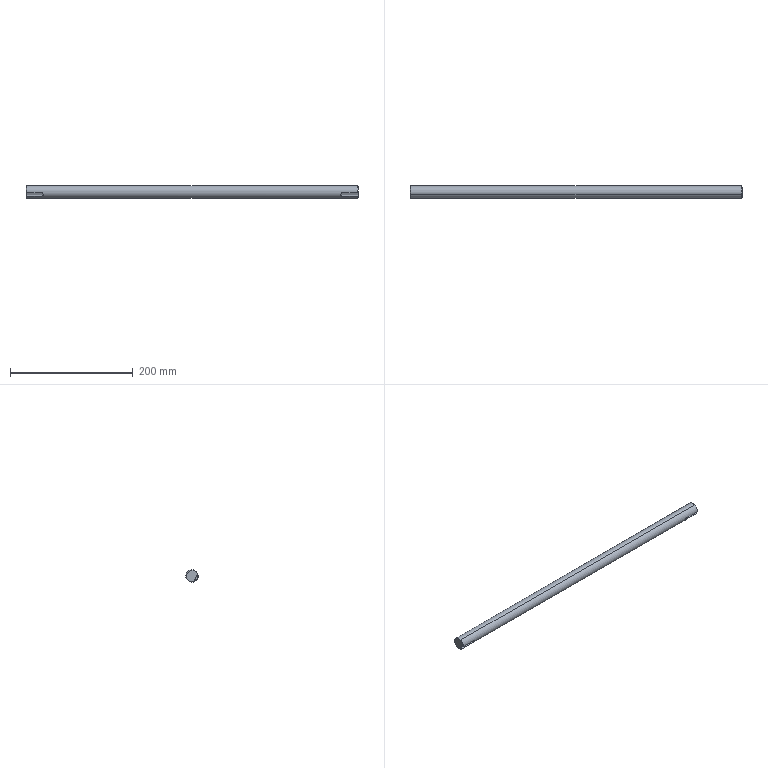Component | SolidWorks | SynchronousAxis-1 | 1 solid | 19 faces | box 540 x 20 x 20 mm | volume 168491 mm3 | plane 8 | cone 6 | cylinder 5 | commonest cylinder face diameters 6 x3 20 x2
build123d program:
from build123d import *

# Parameters (mm, degrees)
SKETCH1_R           = 10
BOSS_EXTRUDE1_DEPTH = 540
CHAMFER1_SIZE       = 1
CUT_EXTRUDE1_DEPTH  = 3.5


with BuildPart() as part:
    # Sketch1 → Boss-Extrude1 (new body)
    with BuildSketch(Plane.XY):
        Circle(SKETCH1_R)
    extrude(amount=BOSS_EXTRUDE1_DEPTH)

    # Chamfer1
    chamfer1_edges = [part.edges().sort_by_distance(p)[0] for p in [
        (-10, 0, 0),
        (-10, 0, 540),
    ]]
    chamfer(chamfer1_edges, length=CHAMFER1_SIZE)

    # Sketch2 → Cut-Extrude1 (cut)
    with BuildSketch(Plane(origin=(0, -10, 0), x_dir=(-1, 0, 0), z_dir=(0, -1, 0))):
        with BuildLine():
            Line((3, 25), (3, -25))
            ThreePointArc((3, -25), (0, -28), (-3, -25))
            Line((-3, -25), (-3, 25))
            ThreePointArc((-3, 25), (0, 28), (3, 25))
        make_face()
    cut_extrude1 = extrude(amount=-CUT_EXTRUDE1_DEPTH, mode=Mode.SUBTRACT)

    # Mirror1: Cut-Extrude1 across plane
    add(cut_extrude1.mirror(Plane.XY.offset(270)), mode=Mode.SUBTRACT)


solid = part.part

# Placed as in the assembly
solid = solid.moved(Location((-244.371, 34.1, 498.836), (24.724, 90, 0)))
STEP:
#1=COLOUR_RGB('',0.7922,0.8196,0.9333);
#2=FILL_AREA_STYLE_COLOUR('',#1);
#3=FILL_AREA_STYLE('',(#2));
#4=SURFACE_STYLE_FILL_AREA(#3);
#5=SURFACE_SIDE_STYLE('',(#4));
#6=SURFACE_STYLE_USAGE(.BOTH.,#5);
#7=PRESENTATION_STYLE_ASSIGNMENT((#6));
#8=CARTESIAN_POINT('',(10.655,1.159,19.425));
#9=VERTEX_POINT('',#8);
#10=CARTESIAN_POINT('',(10.537,1.11,19.532));
#11=VERTEX_POINT('',#10);
#12=CARTESIAN_POINT('',(10.655,1.11,19.532));
#13=DIRECTION('',(-0.,0.9083,0.4182));
#14=DIRECTION('',(1.,0.,0.));
#15=AXIS2_PLACEMENT_3D('',#12,#13,#14);
#16=CIRCLE('',#15,0.1181);
#17=EDGE_CURVE('',#9,#11,#16,.T.);
#18=ORIENTED_EDGE('',*,*,#17,.T.);
#19=CARTESIAN_POINT('',(10.537,0.9849,19.475));
#20=VERTEX_POINT('',#19);
#21=CARTESIAN_POINT('',(10.537,1.11,19.532));
#22=DIRECTION('',(0.,-0.9083,-0.4182));
#23=VECTOR('',#22,39.37);
#24=LINE('',#21,#23);
#25=EDGE_CURVE('',#11,#20,#24,.T.);
#26=ORIENTED_EDGE('',*,*,#25,.T.);
#27=CARTESIAN_POINT('',(10.655,1.051,19.375));
#28=VERTEX_POINT('',#27);
#29=CARTESIAN_POINT('',(10.537,0.9849,19.475));
#30=CARTESIAN_POINT('',(10.537,0.9881,19.467));
#31=CARTESIAN_POINT('',(10.537,0.9917,19.46));
#32=CARTESIAN_POINT('',(10.54,0.9988,19.447));
#33=CARTESIAN_POINT('',(10.543,1.002,19.441));
#34=CARTESIAN_POINT('',(10.549,1.01,19.428));
#35=CARTESIAN_POINT('',(10.552,1.014,19.422));
#36=CARTESIAN_POINT('',(10.561,1.021,19.412));
#37=CARTESIAN_POINT('',(10.566,1.025,19.407));
#38=CARTESIAN_POINT('',(10.577,1.031,19.398));
#39=CARTESIAN_POINT('',(10.583,1.034,19.394));
#40=CARTESIAN_POINT('',(10.595,1.04,19.387));
#41=CARTESIAN_POINT('',(10.602,1.042,19.384));
#42=CARTESIAN_POINT('',(10.616,1.047,19.38));
#43=CARTESIAN_POINT('',(10.624,1.048,19.378));
#44=CARTESIAN_POINT('',(10.639,1.05,19.375));
#45=CARTESIAN_POINT('',(10.647,1.051,19.375));
#46=CARTESIAN_POINT('',(10.655,1.051,19.375));
#47=B_SPLINE_CURVE_WITH_KNOTS('',3,(#29,#30,#31,#32,#33,#34,#35,#36,#37,#38,#39,#40,#41,#42,#43,#44,#45,#46),.UNSPECIFIED.,.F.,.F.,(4,2,2,2,2,2,2,2,4),(0.004718,0.005307,0.005896,0.006485,0.007074,0.007663,0.008252,0.008842,0.009431),.UNSPECIFIED.);
#48=EDGE_CURVE('',#20,#28,#47,.T.);
#49=ORIENTED_EDGE('',*,*,#48,.T.);
#50=CARTESIAN_POINT('',(10.655,1.159,19.425));
#51=DIRECTION('',(0.,-0.9083,-0.4182));
#52=VECTOR('',#51,39.37);
#53=LINE('',#50,#52);
#54=EDGE_CURVE('',#9,#28,#53,.T.);
#55=ORIENTED_EDGE('',*,*,#54,.F.);
#56=EDGE_LOOP('',(#18,#26,#49,#55));
#57=FACE_OUTER_BOUND('',#56,.T.);
#58=CARTESIAN_POINT('',(10.655,1.11,19.532));
#59=DIRECTION('',(0.,-0.9083,-0.4182));
#60=DIRECTION('',(-1.,-0.,0.));
#61=AXIS2_PLACEMENT_3D('',#58,#59,#60);
#62=CYLINDRICAL_SURFACE('',#61,0.1181);
#63=ADVANCED_FACE('',(#57),#62,.F.);
#64=CARTESIAN_POINT('',(-9.621,1.194,19.961));
#65=VERTEX_POINT('',#64);
#66=CARTESIAN_POINT('',(-9.621,1.491,19.317));
#67=VERTEX_POINT('',#66);
#68=CARTESIAN_POINT('',(-9.621,1.343,19.639));
#69=DIRECTION('',(-1.,-0.,0.));
#70=DIRECTION('',(-0.,0.4182,-0.9083));
#71=AXIS2_PLACEMENT_3D('',#68,#69,#70);
#72=CIRCLE('',#71,0.3543);
#73=EDGE_CURVE('',#65,#67,#72,.T.);
#74=ORIENTED_EDGE('',*,*,#73,.F.);
#75=CARTESIAN_POINT('',(-9.582,1.178,19.997));
#76=VERTEX_POINT('',#75);
#77=CARTESIAN_POINT('',(-9.582,1.178,19.997));
#78=DIRECTION('',(0.7071,-0.2957,0.6423));
#79=VECTOR('',#78,39.37);
#80=LINE('',#77,#79);
#81=EDGE_CURVE('',#65,#76,#80,.T.);
#82=ORIENTED_EDGE('',*,*,#81,.T.);
#83=CARTESIAN_POINT('',(-9.582,1.507,19.282));
#84=VERTEX_POINT('',#83);
#85=CARTESIAN_POINT('',(-9.582,1.343,19.639));
#86=DIRECTION('',(1.,0.,-0.));
#87=DIRECTION('',(-0.,0.4182,-0.9083));
#88=AXIS2_PLACEMENT_3D('',#85,#86,#87);
#89=CIRCLE('',#88,0.3937);
#90=EDGE_CURVE('',#84,#76,#89,.T.);
#91=ORIENTED_EDGE('',*,*,#90,.F.);
#92=CARTESIAN_POINT('',(-9.582,1.507,19.282));
#93=DIRECTION('',(0.7071,0.2957,-0.6423));
#94=VECTOR('',#93,39.37);
#95=LINE('',#92,#94);
#96=EDGE_CURVE('',#67,#84,#95,.T.);
#97=ORIENTED_EDGE('',*,*,#96,.F.);
#98=EDGE_LOOP('',(#74,#82,#91,#97));
#99=FACE_OUTER_BOUND('',#98,.T.);
#100=CARTESIAN_POINT('',(-9.582,1.343,19.639));
#101=DIRECTION('',(1.,0.,-0.));
#102=DIRECTION('',(-0.,0.4182,-0.9083));
#103=AXIS2_PLACEMENT_3D('',#100,#101,#102);
#104=CONICAL_SURFACE('',#103,0.3937,0.7854);
#105=ADVANCED_FACE('',(#99),#104,.T.);
#106=CARTESIAN_POINT('',(-9.621,1.088,19.392));
#107=VERTEX_POINT('',#106);
#108=CARTESIAN_POINT('',(-9.621,1.343,19.639));
#109=DIRECTION('',(-1.,-0.,0.));
#110=DIRECTION('',(-0.,0.4182,-0.9083));
#111=AXIS2_PLACEMENT_3D('',#108,#109,#110);
#112=CIRCLE('',#111,0.3543);
#113=EDGE_CURVE('',#67,#107,#112,.T.);
#114=ORIENTED_EDGE('',*,*,#113,.F.);
#115=ORIENTED_EDGE('',*,*,#96,.T.);
#116=CARTESIAN_POINT('',(-9.582,1.051,19.375));
#117=VERTEX_POINT('',#116);
#118=CARTESIAN_POINT('',(-9.582,1.343,19.639));
#119=DIRECTION('',(1.,0.,-0.));
#120=DIRECTION('',(-0.,0.4182,-0.9083));
#121=AXIS2_PLACEMENT_3D('',#118,#119,#120);
#122=CIRCLE('',#121,0.3937);
#123=EDGE_CURVE('',#117,#84,#122,.T.);
#124=ORIENTED_EDGE('',*,*,#123,.F.);
#125=CARTESIAN_POINT('',(-9.621,1.088,19.392));
#126=CARTESIAN_POINT('',(-9.608,1.076,19.386));
#127=CARTESIAN_POINT('',(-9.595,1.063,19.381));
#128=CARTESIAN_POINT('',(-9.582,1.051,19.375));
#129=B_SPLINE_CURVE_WITH_KNOTS('',3,(#125,#126,#127,#128),.UNSPECIFIED.,.F.,.F.,(4,4),(0.005441,0.006894),.UNSPECIFIED.);
#130=EDGE_CURVE('',#107,#117,#129,.T.);
#131=ORIENTED_EDGE('',*,*,#130,.F.);
#132=EDGE_LOOP('',(#114,#115,#124,#131));
#133=FACE_OUTER_BOUND('',#132,.T.);
#134=CARTESIAN_POINT('',(-9.582,1.343,19.639));
#135=DIRECTION('',(1.,0.,-0.));
#136=DIRECTION('',(-0.,0.4182,-0.9083));
#137=AXIS2_PLACEMENT_3D('',#134,#135,#136);
#138=CONICAL_SURFACE('',#137,0.3937,0.7854);
#139=ADVANCED_FACE('',(#133),#138,.T.);
#140=CARTESIAN_POINT('',(11.639,1.491,19.317));
#141=VERTEX_POINT('',#140);
#142=CARTESIAN_POINT('',(11.639,1.194,19.961));
#143=VERTEX_POINT('',#142);
#144=CARTESIAN_POINT('',(11.639,1.343,19.639));
#145=DIRECTION('',(1.,0.,-0.));
#146=DIRECTION('',(0.,0.4182,-0.9083));
#147=AXIS2_PLACEMENT_3D('',#144,#145,#146);
#148=CIRCLE('',#147,0.3543);
#149=EDGE_CURVE('',#141,#143,#148,.T.);
#150=ORIENTED_EDGE('',*,*,#149,.F.);
#151=CARTESIAN_POINT('',(11.6,1.507,19.282));
#152=VERTEX_POINT('',#151);
#153=CARTESIAN_POINT('',(11.639,1.491,19.317));
#154=DIRECTION('',(-0.7071,0.2957,-0.6423));
#155=VECTOR('',#154,39.37);
#156=LINE('',#153,#155);
#157=EDGE_CURVE('',#141,#152,#156,.T.);
#158=ORIENTED_EDGE('',*,*,#157,.T.);
#159=CARTESIAN_POINT('',(11.6,1.178,19.997));
#160=VERTEX_POINT('',#159);
#161=CARTESIAN_POINT('',(11.6,1.343,19.639));
#162=DIRECTION('',(-1.,-0.,0.));
#163=DIRECTION('',(0.,0.4182,-0.9083));
#164=AXIS2_PLACEMENT_3D('',#161,#162,#163);
#165=CIRCLE('',#164,0.3937);
#166=EDGE_CURVE('',#160,#152,#165,.T.);
#167=ORIENTED_EDGE('',*,*,#166,.F.);
#168=CARTESIAN_POINT('',(11.639,1.194,19.961));
#169=DIRECTION('',(-0.7071,-0.2957,0.6423));
#170=VECTOR('',#169,39.37);
#171=LINE('',#168,#170);
#172=EDGE_CURVE('',#143,#160,#171,.T.);
#173=ORIENTED_EDGE('',*,*,#172,.F.);
#174=EDGE_LOOP('',(#150,#158,#167,#173));
#175=FACE_OUTER_BOUND('',#174,.T.);
#176=CARTESIAN_POINT('',(11.639,1.343,19.639));
#177=DIRECTION('',(-1.,-0.,0.));
#178=DIRECTION('',(0.,-0.4182,0.9083));
#179=AXIS2_PLACEMENT_3D('',#176,#177,#178);
#180=CONICAL_SURFACE('',#179,0.3543,0.7854);
#181=ADVANCED_FACE('',(#175),#180,.T.);
#182=CARTESIAN_POINT('',(11.639,0.9897,19.607));
#183=VERTEX_POINT('',#182);
#184=CARTESIAN_POINT('',(11.639,1.343,19.639));
#185=DIRECTION('',(1.,0.,-0.));
#186=DIRECTION('',(0.,0.4182,-0.9083));
#187=AXIS2_PLACEMENT_3D('',#184,#185,#186);
#188=CIRCLE('',#187,0.3543);
#189=EDGE_CURVE('',#143,#183,#188,.T.);
#190=ORIENTED_EDGE('',*,*,#189,.F.);
#191=ORIENTED_EDGE('',*,*,#172,.T.);
#192=CARTESIAN_POINT('',(11.6,0.952,19.589));
#193=VERTEX_POINT('',#192);
#194=CARTESIAN_POINT('',(11.6,1.343,19.639));
#195=DIRECTION('',(-1.,-0.,0.));
#196=DIRECTION('',(0.,0.4182,-0.9083));
#197=AXIS2_PLACEMENT_3D('',#194,#195,#196);
#198=CIRCLE('',#197,0.3937);
#199=EDGE_CURVE('',#193,#160,#198,.T.);
#200=ORIENTED_EDGE('',*,*,#199,.F.);
#201=CARTESIAN_POINT('',(11.6,0.952,19.589));
#202=CARTESIAN_POINT('',(11.613,0.9645,19.595));
#203=CARTESIAN_POINT('',(11.626,0.9771,19.601));
#204=CARTESIAN_POINT('',(11.639,0.9897,19.607));
#205=B_SPLINE_CURVE_WITH_KNOTS('',3,(#201,#202,#203,#204),.UNSPECIFIED.,.F.,.F.,(4,4),(0.005238,0.006691),.UNSPECIFIED.);
#206=EDGE_CURVE('',#193,#183,#205,.T.);
#207=ORIENTED_EDGE('',*,*,#206,.T.);
#208=EDGE_LOOP('',(#190,#191,#200,#207));
#209=FACE_OUTER_BOUND('',#208,.T.);
#210=CARTESIAN_POINT('',(11.639,1.343,19.639));
#211=DIRECTION('',(-1.,-0.,0.));
#212=DIRECTION('',(0.,-0.4182,0.9083));
#213=AXIS2_PLACEMENT_3D('',#210,#211,#212);
#214=CONICAL_SURFACE('',#213,0.3543,0.7854);
#215=ADVANCED_FACE('',(#209),#214,.T.);
#216=ORIENTED_EDGE('',*,*,#166,.T.);
#217=CARTESIAN_POINT('',(11.639,1.507,19.282));
#218=DIRECTION('',(-1.,-0.,0.));
#219=VECTOR('',#218,39.37);
#220=LINE('',#217,#219);
#221=EDGE_CURVE('',#152,#84,#220,.T.);
#222=ORIENTED_EDGE('',*,*,#221,.T.);
#223=ORIENTED_EDGE('',*,*,#90,.T.);
#224=CARTESIAN_POINT('',(11.639,1.178,19.997));
#225=DIRECTION('',(-1.,-0.,0.));
#226=VECTOR('',#225,39.37);
#227=LINE('',#224,#226);
#228=EDGE_CURVE('',#160,#76,#227,.T.);
#229=ORIENTED_EDGE('',*,*,#228,.F.);
#230=EDGE_LOOP('',(#216,#222,#223,#229));
#231=FACE_OUTER_BOUND('',#230,.T.);
#232=CARTESIAN_POINT('',(11.639,1.343,19.639));
#233=DIRECTION('',(-1.,-0.,0.));
#234=DIRECTION('',(0.,-0.4182,0.9083));
#235=AXIS2_PLACEMENT_3D('',#232,#233,#234);
#236=CYLINDRICAL_SURFACE('',#235,0.3937);
#237=ADVANCED_FACE('',(#231),#236,.T.);
#238=ORIENTED_EDGE('',*,*,#221,.F.);
#239=CARTESIAN_POINT('',(11.6,1.051,19.375));
#240=VERTEX_POINT('',#239);
#241=CARTESIAN_POINT('',(11.6,1.343,19.639));
#242=DIRECTION('',(-1.,-0.,0.));
#243=DIRECTION('',(0.,0.4182,-0.9083));
#244=AXIS2_PLACEMENT_3D('',#241,#242,#243);
#245=CIRCLE('',#244,0.3937);
#246=EDGE_CURVE('',#152,#240,#245,.T.);
#247=ORIENTED_EDGE('',*,*,#246,.T.);
#248=CARTESIAN_POINT('',(11.639,1.051,19.375));
#249=DIRECTION('',(1.,0.,-0.));
#250=VECTOR('',#249,39.37);
#251=LINE('',#248,#250);
#252=EDGE_CURVE('',#28,#240,#251,.T.);
#253=ORIENTED_EDGE('',*,*,#252,.F.);
#254=ORIENTED_EDGE('',*,*,#48,.F.);
#255=CARTESIAN_POINT('',(10.655,0.952,19.589));
#256=VERTEX_POINT('',#255);
#257=CARTESIAN_POINT('',(10.655,0.952,19.589));
#258=CARTESIAN_POINT('',(10.647,0.952,19.589));
#259=CARTESIAN_POINT('',(10.639,0.9521,19.589));
#260=CARTESIAN_POINT('',(10.624,0.9525,19.585));
#261=CARTESIAN_POINT('',(10.616,0.9528,19.583));
#262=CARTESIAN_POINT('',(10.602,0.9538,19.577));
#263=CARTESIAN_POINT('',(10.595,0.9544,19.573));
#264=CARTESIAN_POINT('',(10.583,0.9559,19.565));
#265=CARTESIAN_POINT('',(10.577,0.9569,19.56));
#266=CARTESIAN_POINT('',(10.56,0.9605,19.543));
#267=CARTESIAN_POINT('',(10.552,0.9639,19.53));
#268=CARTESIAN_POINT('',(10.543,0.9705,19.51));
#269=CARTESIAN_POINT('',(10.54,0.9731,19.503));
#270=CARTESIAN_POINT('',(10.537,0.9786,19.489));
#271=CARTESIAN_POINT('',(10.537,0.9817,19.482));
#272=CARTESIAN_POINT('',(10.537,0.9849,19.475));
#273=B_SPLINE_CURVE_WITH_KNOTS('',3,(#257,#258,#259,#260,#261,#262,#263,#264,#265,#266,#267,#268,#269,#270,#271,#272),.UNSPECIFIED.,.F.,.F.,(4,2,2,2,2,2,2,4),(0.,0.0005898,0.00118,0.001769,0.002359,0.003539,0.004128,0.004718),.UNSPECIFIED.);
#274=EDGE_CURVE('',#256,#20,#273,.T.);
#275=ORIENTED_EDGE('',*,*,#274,.F.);
#276=CARTESIAN_POINT('',(11.639,0.952,19.589));
#277=DIRECTION('',(-1.,-0.,0.));
#278=VECTOR('',#277,39.37);
#279=LINE('',#276,#278);
#280=EDGE_CURVE('',#193,#256,#279,.T.);
#281=ORIENTED_EDGE('',*,*,#280,.F.);
#282=ORIENTED_EDGE('',*,*,#199,.T.);
#283=ORIENTED_EDGE('',*,*,#228,.T.);
#284=CARTESIAN_POINT('',(-9.582,0.952,19.589));
#285=VERTEX_POINT('',#284);
#286=CARTESIAN_POINT('',(-9.582,1.343,19.639));
#287=DIRECTION('',(1.,0.,-0.));
#288=DIRECTION('',(-0.,0.4182,-0.9083));
#289=AXIS2_PLACEMENT_3D('',#286,#287,#288);
#290=CIRCLE('',#289,0.3937);
#291=EDGE_CURVE('',#76,#285,#290,.T.);
#292=ORIENTED_EDGE('',*,*,#291,.T.);
#293=CARTESIAN_POINT('',(-8.637,0.952,19.589));
#294=VERTEX_POINT('',#293);
#295=CARTESIAN_POINT('',(11.639,0.952,19.589));
#296=DIRECTION('',(1.,0.,-0.));
#297=VECTOR('',#296,39.37);
#298=LINE('',#295,#297);
#299=EDGE_CURVE('',#285,#294,#298,.T.);
#300=ORIENTED_EDGE('',*,*,#299,.T.);
#301=CARTESIAN_POINT('',(-8.637,1.051,19.375));
#302=VERTEX_POINT('',#301);
#303=CARTESIAN_POINT('',(-8.637,0.952,19.589));
#304=CARTESIAN_POINT('',(-8.629,0.952,19.589));
#305=CARTESIAN_POINT('',(-8.621,0.9521,19.589));
#306=CARTESIAN_POINT('',(-8.606,0.9525,19.585));
#307=CARTESIAN_POINT('',(-8.598,0.9528,19.583));
#308=CARTESIAN_POINT('',(-8.584,0.9538,19.577));
#309=CARTESIAN_POINT('',(-8.577,0.9544,19.573));
#310=CARTESIAN_POINT('',(-8.565,0.9559,19.565));
#311=CARTESIAN_POINT('',(-8.559,0.9569,19.56));
#312=CARTESIAN_POINT('',(-8.542,0.9605,19.543));
#313=CARTESIAN_POINT('',(-8.534,0.9639,19.53));
#314=CARTESIAN_POINT('',(-8.525,0.9705,19.51));
#315=CARTESIAN_POINT('',(-8.522,0.973,19.503));
#316=CARTESIAN_POINT('',(-8.519,0.9786,19.489));
#317=CARTESIAN_POINT('',(-8.519,0.9816,19.482));
#318=CARTESIAN_POINT('',(-8.519,0.9881,19.468));
#319=CARTESIAN_POINT('',(-8.519,0.9916,19.461));
#320=CARTESIAN_POINT('',(-8.522,0.9988,19.447));
#321=CARTESIAN_POINT('',(-8.525,1.002,19.441));
#322=CARTESIAN_POINT('',(-8.531,1.01,19.428));
#323=CARTESIAN_POINT('',(-8.534,1.014,19.423));
#324=CARTESIAN_POINT('',(-8.543,1.021,19.412));
#325=CARTESIAN_POINT('',(-8.548,1.025,19.407));
#326=CARTESIAN_POINT('',(-8.559,1.031,19.398));
#327=CARTESIAN_POINT('',(-8.564,1.034,19.394));
#328=CARTESIAN_POINT('',(-8.577,1.04,19.387));
#329=CARTESIAN_POINT('',(-8.584,1.042,19.384));
#330=CARTESIAN_POINT('',(-8.598,1.047,19.38));
#331=CARTESIAN_POINT('',(-8.606,1.048,19.378));
#332=CARTESIAN_POINT('',(-8.621,1.05,19.375));
#333=CARTESIAN_POINT('',(-8.629,1.051,19.375));
#334=CARTESIAN_POINT('',(-8.637,1.051,19.375));
#335=B_SPLINE_CURVE_WITH_KNOTS('',3,(#303,#304,#305,#306,#307,#308,#309,#310,#311,#312,#313,#314,#315,#316,#317,#318,#319,#320,#321,#322,#323,#324,#325,#326,#327,#328,#329,#330,#331,#332,#333,#334),.UNSPECIFIED.,.F.,.F.,(4,2,2,2,2,2,2,2,2,2,2,2,2,2,2,4),(0.,0.0005894,0.001179,0.001768,0.002358,0.003536,0.004126,0.004715,0.005305,0.005894,0.006484,0.007073,0.007662,0.008252,0.008841,0.009431),.UNSPECIFIED.);
#336=EDGE_CURVE('',#294,#302,#335,.T.);
#337=ORIENTED_EDGE('',*,*,#336,.T.);
#338=CARTESIAN_POINT('',(11.639,1.051,19.375));
#339=DIRECTION('',(-1.,-0.,0.));
#340=VECTOR('',#339,39.37);
#341=LINE('',#338,#340);
#342=EDGE_CURVE('',#302,#117,#341,.T.);
#343=ORIENTED_EDGE('',*,*,#342,.T.);
#344=ORIENTED_EDGE('',*,*,#123,.T.);
#345=EDGE_LOOP('',(#238,#247,#253,#254,#275,#281,#282,#283,#292,#300,#337,#343,#344));
#346=FACE_OUTER_BOUND('',#345,.T.);
#347=CARTESIAN_POINT('',(11.639,1.343,19.639));
#348=DIRECTION('',(-1.,-0.,0.));
#349=DIRECTION('',(0.,-0.4182,0.9083));
#350=AXIS2_PLACEMENT_3D('',#347,#348,#349);
#351=CYLINDRICAL_SURFACE('',#350,0.3937);
#352=ADVANCED_FACE('',(#346),#351,.T.);
#353=CARTESIAN_POINT('',(11.639,1.061,19.639));
#354=VERTEX_POINT('',#353);
#355=CARTESIAN_POINT('',(11.639,1.159,19.425));
#356=VERTEX_POINT('',#355);
#357=CARTESIAN_POINT('',(11.639,1.11,19.532));
#358=DIRECTION('',(-0.,0.4182,-0.9083));
#359=VECTOR('',#358,39.37);
#360=LINE('',#357,#359);
#361=EDGE_CURVE('',#354,#356,#360,.T.);
#362=ORIENTED_EDGE('',*,*,#361,.T.);
#363=CARTESIAN_POINT('',(11.639,1.088,19.392));
#364=VERTEX_POINT('',#363);
#365=CARTESIAN_POINT('',(11.639,1.392,19.532));
#366=DIRECTION('',(0.,-0.9083,-0.4182));
#367=VECTOR('',#366,39.37);
#368=LINE('',#365,#367);
#369=EDGE_CURVE('',#356,#364,#368,.T.);
#370=ORIENTED_EDGE('',*,*,#369,.T.);
#371=CARTESIAN_POINT('',(11.639,1.343,19.639));
#372=DIRECTION('',(1.,0.,-0.));
#373=DIRECTION('',(0.,0.4182,-0.9083));
#374=AXIS2_PLACEMENT_3D('',#371,#372,#373);
#375=CIRCLE('',#374,0.3543);
#376=EDGE_CURVE('',#364,#141,#375,.T.);
#377=ORIENTED_EDGE('',*,*,#376,.T.);
#378=ORIENTED_EDGE('',*,*,#149,.T.);
#379=ORIENTED_EDGE('',*,*,#189,.T.);
#380=CARTESIAN_POINT('',(11.639,1.293,19.746));
#381=DIRECTION('',(-0.,0.9083,0.4182));
#382=VECTOR('',#381,39.37);
#383=LINE('',#380,#382);
#384=EDGE_CURVE('',#183,#354,#383,.T.);
#385=ORIENTED_EDGE('',*,*,#384,.T.);
#386=EDGE_LOOP('',(#362,#370,#377,#378,#379,#385));
#387=FACE_OUTER_BOUND('',#386,.T.);
#388=CARTESIAN_POINT('',(11.639,1.343,19.639));
#389=DIRECTION('',(1.,0.,-0.));
#390=DIRECTION('',(-0.,0.4182,-0.9083));
#391=AXIS2_PLACEMENT_3D('',#388,#389,#390);
#392=PLANE('',#391);
#393=ADVANCED_FACE('',(#387),#392,.T.);
#394=ORIENTED_EDGE('',*,*,#157,.F.);
#395=ORIENTED_EDGE('',*,*,#376,.F.);
#396=CARTESIAN_POINT('',(11.639,1.088,19.392));
#397=CARTESIAN_POINT('',(11.626,1.076,19.386));
#398=CARTESIAN_POINT('',(11.613,1.063,19.381));
#399=CARTESIAN_POINT('',(11.6,1.051,19.375));
#400=B_SPLINE_CURVE_WITH_KNOTS('',3,(#396,#397,#398,#399),.UNSPECIFIED.,.F.,.F.,(4,4),(0.005441,0.006894),.UNSPECIFIED.);
#401=EDGE_CURVE('',#364,#240,#400,.T.);
#402=ORIENTED_EDGE('',*,*,#401,.T.);
#403=ORIENTED_EDGE('',*,*,#246,.F.);
#404=EDGE_LOOP('',(#394,#395,#402,#403));
#405=FACE_OUTER_BOUND('',#404,.T.);
#406=CARTESIAN_POINT('',(11.639,1.343,19.639));
#407=DIRECTION('',(-1.,-0.,0.));
#408=DIRECTION('',(0.,-0.4182,0.9083));
#409=AXIS2_PLACEMENT_3D('',#406,#407,#408);
#410=CONICAL_SURFACE('',#409,0.3543,0.7854);
#411=ADVANCED_FACE('',(#405),#410,.T.);
#412=CARTESIAN_POINT('',(-9.621,1.061,19.639));
#413=VERTEX_POINT('',#412);
#414=CARTESIAN_POINT('',(-9.621,1.159,19.425));
#415=VERTEX_POINT('',#414);
#416=CARTESIAN_POINT('',(-9.621,1.11,19.532));
#417=DIRECTION('',(-0.,0.4182,-0.9083));
#418=VECTOR('',#417,39.37);
#419=LINE('',#416,#418);
#420=EDGE_CURVE('',#413,#415,#419,.T.);
#421=ORIENTED_EDGE('',*,*,#420,.F.);
#422=CARTESIAN_POINT('',(-9.621,0.9897,19.607));
#423=VERTEX_POINT('',#422);
#424=CARTESIAN_POINT('',(-9.621,1.293,19.746));
#425=DIRECTION('',(0.,-0.9083,-0.4182));
#426=VECTOR('',#425,39.37);
#427=LINE('',#424,#426);
#428=EDGE_CURVE('',#413,#423,#427,.T.);
#429=ORIENTED_EDGE('',*,*,#428,.T.);
#430=CARTESIAN_POINT('',(-9.621,1.343,19.639));
#431=DIRECTION('',(-1.,-0.,0.));
#432=DIRECTION('',(-0.,0.4182,-0.9083));
#433=AXIS2_PLACEMENT_3D('',#430,#431,#432);
#434=CIRCLE('',#433,0.3543);
#435=EDGE_CURVE('',#423,#65,#434,.T.);
#436=ORIENTED_EDGE('',*,*,#435,.T.);
#437=ORIENTED_EDGE('',*,*,#73,.T.);
#438=ORIENTED_EDGE('',*,*,#113,.T.);
#439=CARTESIAN_POINT('',(-9.621,1.392,19.532));
#440=DIRECTION('',(-0.,0.9083,0.4182));
#441=VECTOR('',#440,39.37);
#442=LINE('',#439,#441);
#443=EDGE_CURVE('',#107,#415,#442,.T.);
#444=ORIENTED_EDGE('',*,*,#443,.T.);
#445=EDGE_LOOP('',(#421,#429,#436,#437,#438,#444));
#446=FACE_OUTER_BOUND('',#445,.T.);
#447=CARTESIAN_POINT('',(-9.621,1.343,19.639));
#448=DIRECTION('',(1.,0.,-0.));
#449=DIRECTION('',(-0.,0.4182,-0.9083));
#450=AXIS2_PLACEMENT_3D('',#447,#448,#449);
#451=PLANE('',#450);
#452=ADVANCED_FACE('',(#446),#451,.F.);
#453=ORIENTED_EDGE('',*,*,#81,.F.);
#454=ORIENTED_EDGE('',*,*,#435,.F.);
#455=CARTESIAN_POINT('',(-9.582,0.952,19.589));
#456=CARTESIAN_POINT('',(-9.595,0.9645,19.595));
#457=CARTESIAN_POINT('',(-9.608,0.9771,19.601));
#458=CARTESIAN_POINT('',(-9.621,0.9897,19.607));
#459=B_SPLINE_CURVE_WITH_KNOTS('',3,(#455,#456,#457,#458),.UNSPECIFIED.,.F.,.F.,(4,4),(0.005238,0.006691),.UNSPECIFIED.);
#460=EDGE_CURVE('',#285,#423,#459,.T.);
#461=ORIENTED_EDGE('',*,*,#460,.F.);
#462=ORIENTED_EDGE('',*,*,#291,.F.);
#463=EDGE_LOOP('',(#453,#454,#461,#462));
#464=FACE_OUTER_BOUND('',#463,.T.);
#465=CARTESIAN_POINT('',(-9.582,1.343,19.639));
#466=DIRECTION('',(1.,0.,-0.));
#467=DIRECTION('',(-0.,0.4182,-0.9083));
#468=AXIS2_PLACEMENT_3D('',#465,#466,#467);
#469=CONICAL_SURFACE('',#468,0.3937,0.7854);
#470=ADVANCED_FACE('',(#464),#469,.T.);
#471=CARTESIAN_POINT('',(-8.637,1.061,19.639));
#472=VERTEX_POINT('',#471);
#473=CARTESIAN_POINT('',(-8.637,1.061,19.639));
#474=DIRECTION('',(0.,-0.9083,-0.4182));
#475=VECTOR('',#474,39.37);
#476=LINE('',#473,#475);
#477=EDGE_CURVE('',#472,#294,#476,.T.);
#478=ORIENTED_EDGE('',*,*,#477,.F.);
#479=CARTESIAN_POINT('',(-8.637,1.159,19.425));
#480=VERTEX_POINT('',#479);
#481=CARTESIAN_POINT('',(-8.637,1.11,19.532));
#482=DIRECTION('',(0.,-0.9083,-0.4182));
#483=DIRECTION('',(-1.,-0.,0.));
#484=AXIS2_PLACEMENT_3D('',#481,#482,#483);
#485=CIRCLE('',#484,0.1181);
#486=EDGE_CURVE('',#480,#472,#485,.T.);
#487=ORIENTED_EDGE('',*,*,#486,.F.);
#488=CARTESIAN_POINT('',(-8.637,1.159,19.425));
#489=DIRECTION('',(0.,-0.9083,-0.4182));
#490=VECTOR('',#489,39.37);
#491=LINE('',#488,#490);
#492=EDGE_CURVE('',#480,#302,#491,.T.);
#493=ORIENTED_EDGE('',*,*,#492,.T.);
#494=ORIENTED_EDGE('',*,*,#336,.F.);
#495=EDGE_LOOP('',(#478,#487,#493,#494));
#496=FACE_OUTER_BOUND('',#495,.T.);
#497=CARTESIAN_POINT('',(-8.637,1.11,19.532));
#498=DIRECTION('',(0.,-0.9083,-0.4182));
#499=DIRECTION('',(-1.,-0.,0.));
#500=AXIS2_PLACEMENT_3D('',#497,#498,#499);
#501=CYLINDRICAL_SURFACE('',#500,0.1181);
#502=ADVANCED_FACE('',(#496),#501,.F.);
#503=ORIENTED_EDGE('',*,*,#420,.T.);
#504=CARTESIAN_POINT('',(-10.605,1.159,19.425));
#505=DIRECTION('',(1.,0.,0.));
#506=VECTOR('',#505,39.37);
#507=LINE('',#504,#506);
#508=EDGE_CURVE('',#415,#480,#507,.T.);
#509=ORIENTED_EDGE('',*,*,#508,.T.);
#510=ORIENTED_EDGE('',*,*,#486,.T.);
#511=CARTESIAN_POINT('',(-10.605,1.061,19.639));
#512=DIRECTION('',(-1.,-0.,-0.));
#513=VECTOR('',#512,39.37);
#514=LINE('',#511,#513);
#515=EDGE_CURVE('',#472,#413,#514,.T.);
#516=ORIENTED_EDGE('',*,*,#515,.T.);
#517=EDGE_LOOP('',(#503,#509,#510,#516));
#518=FACE_OUTER_BOUND('',#517,.T.);
#519=CARTESIAN_POINT('',(-10.605,1.11,19.532));
#520=DIRECTION('',(0.,-0.9083,-0.4182));
#521=DIRECTION('',(-1.,-0.,0.));
#522=AXIS2_PLACEMENT_3D('',#519,#520,#521);
#523=PLANE('',#522);
#524=ADVANCED_FACE('',(#518),#523,.T.);
#525=ORIENTED_EDGE('',*,*,#460,.T.);
#526=ORIENTED_EDGE('',*,*,#428,.F.);
#527=ORIENTED_EDGE('',*,*,#515,.F.);
#528=ORIENTED_EDGE('',*,*,#477,.T.);
#529=ORIENTED_EDGE('',*,*,#299,.F.);
#530=EDGE_LOOP('',(#525,#526,#527,#528,#529));
#531=FACE_OUTER_BOUND('',#530,.T.);
#532=CARTESIAN_POINT('',(-10.605,1.061,19.639));
#533=DIRECTION('',(0.,-0.4182,0.9083));
#534=DIRECTION('',(1.,0.,0.));
#535=AXIS2_PLACEMENT_3D('',#532,#533,#534);
#536=PLANE('',#535);
#537=ADVANCED_FACE('',(#531),#536,.F.);
#538=ORIENTED_EDGE('',*,*,#492,.F.);
#539=ORIENTED_EDGE('',*,*,#508,.F.);
#540=ORIENTED_EDGE('',*,*,#443,.F.);
#541=ORIENTED_EDGE('',*,*,#130,.T.);
#542=ORIENTED_EDGE('',*,*,#342,.F.);
#543=EDGE_LOOP('',(#538,#539,#540,#541,#542));
#544=FACE_OUTER_BOUND('',#543,.T.);
#545=CARTESIAN_POINT('',(-10.605,1.159,19.425));
#546=DIRECTION('',(-0.,0.4182,-0.9083));
#547=DIRECTION('',(-1.,-0.,-0.));
#548=AXIS2_PLACEMENT_3D('',#545,#546,#547);
#549=PLANE('',#548);
#550=ADVANCED_FACE('',(#544),#549,.F.);
#551=ORIENTED_EDGE('',*,*,#25,.F.);
#552=CARTESIAN_POINT('',(10.655,1.061,19.639));
#553=VERTEX_POINT('',#552);
#554=CARTESIAN_POINT('',(10.655,1.11,19.532));
#555=DIRECTION('',(-0.,0.9083,0.4182));
#556=DIRECTION('',(1.,0.,0.));
#557=AXIS2_PLACEMENT_3D('',#554,#555,#556);
#558=CIRCLE('',#557,0.1181);
#559=EDGE_CURVE('',#11,#553,#558,.T.);
#560=ORIENTED_EDGE('',*,*,#559,.T.);
#561=CARTESIAN_POINT('',(10.655,1.061,19.639));
#562=DIRECTION('',(0.,-0.9083,-0.4182));
#563=VECTOR('',#562,39.37);
#564=LINE('',#561,#563);
#565=EDGE_CURVE('',#553,#256,#564,.T.);
#566=ORIENTED_EDGE('',*,*,#565,.T.);
#567=ORIENTED_EDGE('',*,*,#274,.T.);
#568=EDGE_LOOP('',(#551,#560,#566,#567));
#569=FACE_OUTER_BOUND('',#568,.T.);
#570=CARTESIAN_POINT('',(10.655,1.11,19.532));
#571=DIRECTION('',(0.,-0.9083,-0.4182));
#572=DIRECTION('',(-1.,-0.,0.));
#573=AXIS2_PLACEMENT_3D('',#570,#571,#572);
#574=CYLINDRICAL_SURFACE('',#573,0.1181);
#575=ADVANCED_FACE('',(#569),#574,.F.);
#576=ORIENTED_EDGE('',*,*,#252,.T.);
#577=ORIENTED_EDGE('',*,*,#401,.F.);
#578=ORIENTED_EDGE('',*,*,#369,.F.);
#579=CARTESIAN_POINT('',(12.623,1.159,19.425));
#580=DIRECTION('',(-1.,-0.,0.));
#581=VECTOR('',#580,39.37);
#582=LINE('',#579,#581);
#583=EDGE_CURVE('',#356,#9,#582,.T.);
#584=ORIENTED_EDGE('',*,*,#583,.T.);
#585=ORIENTED_EDGE('',*,*,#54,.T.);
#586=EDGE_LOOP('',(#576,#577,#578,#584,#585));
#587=FACE_OUTER_BOUND('',#586,.T.);
#588=CARTESIAN_POINT('',(12.623,1.159,19.425));
#589=DIRECTION('',(0.,-0.4182,0.9083));
#590=DIRECTION('',(1.,0.,-0.));
#591=AXIS2_PLACEMENT_3D('',#588,#589,#590);
#592=PLANE('',#591);
#593=ADVANCED_FACE('',(#587),#592,.T.);
#594=ORIENTED_EDGE('',*,*,#280,.T.);
#595=ORIENTED_EDGE('',*,*,#565,.F.);
#596=CARTESIAN_POINT('',(12.623,1.061,19.639));
#597=DIRECTION('',(1.,0.,-0.));
#598=VECTOR('',#597,39.37);
#599=LINE('',#596,#598);
#600=EDGE_CURVE('',#553,#354,#599,.T.);
#601=ORIENTED_EDGE('',*,*,#600,.T.);
#602=ORIENTED_EDGE('',*,*,#384,.F.);
#603=ORIENTED_EDGE('',*,*,#206,.F.);
#604=EDGE_LOOP('',(#594,#595,#601,#602,#603));
#605=FACE_OUTER_BOUND('',#604,.T.);
#606=CARTESIAN_POINT('',(12.623,1.061,19.639));
#607=DIRECTION('',(-0.,0.4182,-0.9083));
#608=DIRECTION('',(-1.,-0.,0.));
#609=AXIS2_PLACEMENT_3D('',#606,#607,#608);
#610=PLANE('',#609);
#611=ADVANCED_FACE('',(#605),#610,.T.);
#612=ORIENTED_EDGE('',*,*,#600,.F.);
#613=ORIENTED_EDGE('',*,*,#559,.F.);
#614=ORIENTED_EDGE('',*,*,#17,.F.);
#615=ORIENTED_EDGE('',*,*,#583,.F.);
#616=ORIENTED_EDGE('',*,*,#361,.F.);
#617=EDGE_LOOP('',(#612,#613,#614,#615,#616));
#618=FACE_OUTER_BOUND('',#617,.T.);
#619=CARTESIAN_POINT('',(12.623,1.11,19.532));
#620=DIRECTION('',(0.,-0.9083,-0.4182));
#621=DIRECTION('',(1.,0.,-0.));
#622=AXIS2_PLACEMENT_3D('',#619,#620,#621);
#623=PLANE('',#622);
#624=ADVANCED_FACE('',(#618),#623,.T.);
#625=CLOSED_SHELL('',(#63,#105,#139,#181,#215,#237,#352,#393,#411,#452,#470,#502,#524,#537,#550,#575,#593,#611,#624));
#626=MANIFOLD_SOLID_BREP('',#625);
#627=STYLED_ITEM('',(#7),#626);
#628=PRESENTATION_LAYER_ASSIGNMENT('','',(#627));
#629=CARTESIAN_POINT('',(0.,0.,0.));
#630=DIRECTION('',(0.,0.,1.));
#631=DIRECTION('',(1.,0.,0.));
#632=AXIS2_PLACEMENT_3D('',#629,#630,#631);
#633=(LENGTH_UNIT()NAMED_UNIT(*)SI_UNIT($,.METRE.));
#634=LENGTH_MEASURE_WITH_UNIT(LENGTH_MEASURE(0.0254),#633);
#635=DIMENSIONAL_EXPONENTS(1.,0.,0.,0.,0.,0.,0.);
#636=(CONVERSION_BASED_UNIT('',#634)LENGTH_UNIT()NAMED_UNIT(#635));
#637=UNCERTAINTY_MEASURE_WITH_UNIT(LENGTH_MEASURE(0.00001),#636,'','');
#638=(NAMED_UNIT(*)PLANE_ANGLE_UNIT()SI_UNIT($,.RADIAN.));
#639=(NAMED_UNIT(*)SI_UNIT($,.STERADIAN.)SOLID_ANGLE_UNIT());
#640=(GEOMETRIC_REPRESENTATION_CONTEXT(3)GLOBAL_UNCERTAINTY_ASSIGNED_CONTEXT((#637))GLOBAL_UNIT_ASSIGNED_CONTEXT((#636,#638,#639))REPRESENTATION_CONTEXT('',''));
#641=ADVANCED_BREP_SHAPE_REPRESENTATION('',(#626,#632),#640);
#642=(LENGTH_UNIT()NAMED_UNIT(*)SI_UNIT($,.METRE.));
#643=LENGTH_MEASURE_WITH_UNIT(LENGTH_MEASURE(0.0254),#642);
#644=DIMENSIONAL_EXPONENTS(1.,0.,0.,0.,0.,0.,0.);
#645=(CONVERSION_BASED_UNIT('',#643)LENGTH_UNIT()NAMED_UNIT(#644));
#646=UNCERTAINTY_MEASURE_WITH_UNIT(LENGTH_MEASURE(0.00001),#645,'','');
#647=(NAMED_UNIT(*)PLANE_ANGLE_UNIT()SI_UNIT($,.RADIAN.));
#648=(NAMED_UNIT(*)SI_UNIT($,.STERADIAN.)SOLID_ANGLE_UNIT());
#649=(GEOMETRIC_REPRESENTATION_CONTEXT(3)GLOBAL_UNCERTAINTY_ASSIGNED_CONTEXT((#646))GLOBAL_UNIT_ASSIGNED_CONTEXT((#645,#647,#648))REPRESENTATION_CONTEXT('',''));
#650=MECHANICAL_DESIGN_GEOMETRIC_PRESENTATION_REPRESENTATION('',(#627),#649);